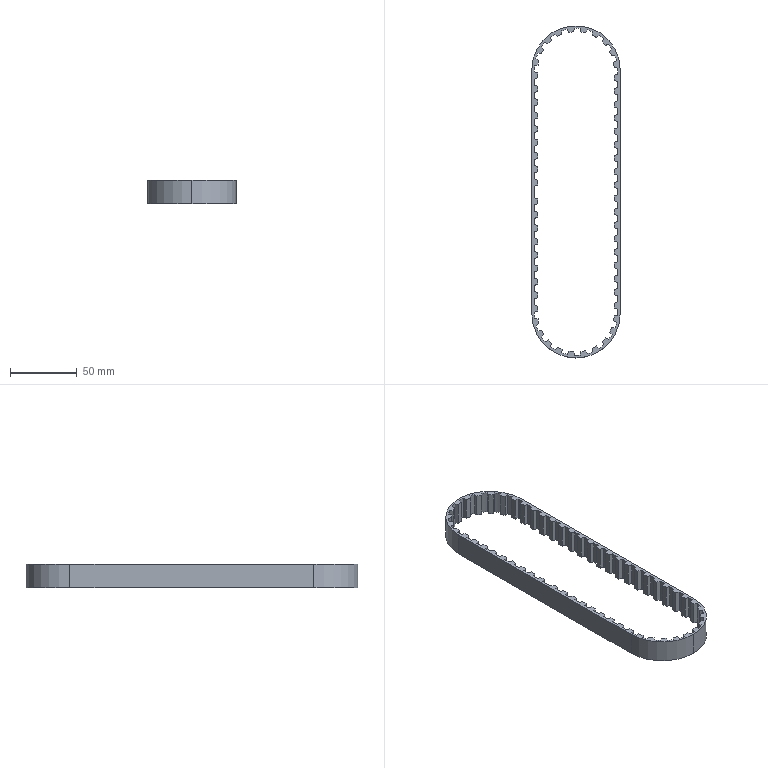Component | SolidWorks | SynchronousBelt-2 | 1 solid | 236 faces | box 66 x 248 x 17.3 mm | volume 30311 mm3 | plane 210 | cylinder 26 | commonest cylinder face diameters 62.1 x23 66 x3
build123d program:
from build123d import *

# Parameters (mm, degrees)
BOSS_EXTRUDE1_DEPTH                        = 17.3
T10_TOOTH_PROFILE_INNER_CONTOUR_DEPTH      = 129.624
T10_TOOTH_PROFILE_INNER_CONTOUR_DEPTH_BACK = 129.624


with BuildPart() as part:
    # Sketch1_2 → Boss-Extrude1 (new body)
    with BuildSketch(Plane.XY.offset(8.4)):
        with BuildLine():
            Line((-91, -33), (91, -33))
            ThreePointArc((91, -33), (124, 0), (91, 33))
            Line((91, 33), (-91, 33))
            ThreePointArc((-91, 33), (-124, 0), (-91, -33))
        make_face()
        with BuildLine():
            Line((-102.801, 22.266), (-102.873, 24.877))
            Line((-102.873, 24.877), (-99.358, 26.267))
            Line((-99.358, 26.267), (-97.625, 24.314))
            ThreePointArc((-97.625, 24.314), (-95.718, 24.754), (-93.783, 25.046))
            Line((-93.783, 25.046), (-92.89, 27.5))
            Line((-92.89, 27.5), (-89.11, 27.5))
            Line((-89.11, 27.5), (-88.273, 25.2))
            Line((-88.273, 25.2), (-82.803, 25.2))
            Line((-82.803, 25.2), (-81.966, 27.5))
            Line((-81.966, 27.5), (-78.186, 27.5))
            Line((-78.186, 27.5), (-77.349, 25.2))
            Line((-77.349, 25.2), (-71.879, 25.2))
            Line((-71.879, 25.2), (-71.042, 27.5))
            Line((-71.042, 27.5), (-67.261, 27.5))
            Line((-67.261, 27.5), (-66.424, 25.2))
            Line((-66.424, 25.2), (-60.954, 25.2))
            Line((-60.954, 25.2), (-60.117, 27.5))
            Line((-60.117, 27.5), (-56.337, 27.5))
            Line((-56.337, 27.5), (-55.5, 25.2))
            Line((-55.5, 25.2), (-50.03, 25.2))
            Line((-50.03, 25.2), (-49.193, 27.5))
            Line((-49.193, 27.5), (-45.413, 27.5))
            Line((-45.413, 27.5), (-44.576, 25.2))
            Line((-44.576, 25.2), (-39.106, 25.2))
            Line((-39.106, 25.2), (-38.269, 27.5))
            Line((-38.269, 27.5), (-34.489, 27.5))
            Line((-34.489, 27.5), (-33.652, 25.2))
            Line((-33.652, 25.2), (-28.182, 25.2))
            Line((-28.182, 25.2), (-27.345, 27.5))
            Line((-27.345, 27.5), (-23.564, 27.5))
            Line((-23.564, 27.5), (-22.727, 25.2))
            Line((-22.727, 25.2), (-17.257, 25.2))
            Line((-17.257, 25.2), (-16.42, 27.5))
            Line((-16.42, 27.5), (-12.64, 27.5))
            Line((-12.64, 27.5), (-11.803, 25.2))
            Line((-11.803, 25.2), (-6.333, 25.2))
            Line((-6.333, 25.2), (-5.496, 27.5))
            Line((-5.496, 27.5), (-1.716, 27.5))
            Line((-1.716, 27.5), (-0.8788, 25.2))
            Line((-0.8788, 25.2), (4.591, 25.2))
            Line((4.591, 25.2), (5.428, 27.5))
            Line((5.428, 27.5), (9.208, 27.5))
            Line((9.208, 27.5), (10.045, 25.2))
            Line((10.045, 25.2), (15.515, 25.2))
            Line((15.515, 25.2), (16.352, 27.5))
            Line((16.352, 27.5), (20.133, 27.5))
            Line((20.133, 27.5), (20.97, 25.2))
            Line((20.97, 25.2), (26.44, 25.2))
            Line((26.44, 25.2), (27.277, 27.5))
            Line((27.277, 27.5), (31.057, 27.5))
            Line((31.057, 27.5), (31.894, 25.2))
            Line((31.894, 25.2), (37.364, 25.2))
            Line((37.364, 25.2), (38.201, 27.5))
            Line((38.201, 27.5), (41.981, 27.5))
            Line((41.981, 27.5), (42.818, 25.2))
            Line((42.818, 25.2), (48.288, 25.2))
            Line((48.288, 25.2), (49.125, 27.5))
            Line((49.125, 27.5), (52.905, 27.5))
            Line((52.905, 27.5), (53.742, 25.2))
            Line((53.742, 25.2), (59.212, 25.2))
            Line((59.212, 25.2), (60.049, 27.5))
            Line((60.049, 27.5), (63.83, 27.5))
            Line((63.83, 27.5), (64.667, 25.2))
            Line((64.667, 25.2), (70.137, 25.2))
            Line((70.137, 25.2), (70.974, 27.5))
            Line((70.974, 27.5), (74.754, 27.5))
            Line((74.754, 27.5), (75.591, 25.2))
            Line((75.591, 25.2), (81.061, 25.2))
            Line((81.061, 25.2), (81.898, 27.5))
            Line((81.898, 27.5), (85.678, 27.5))
            Line((85.678, 27.5), (86.515, 25.2))
            Line((86.515, 25.2), (91, 25.2))
            ThreePointArc((91, 25.2), (91.218, 25.199), (91.437, 25.196))
            Line((91.437, 25.196), (92.636, 27.516))
            Line((92.636, 27.516), (96.385, 27.034))
            Line((96.385, 27.034), (96.958, 24.486))
            ThreePointArc((96.958, 24.486), (98.84, 23.949), (100.675, 23.269))
            Line((100.675, 23.269), (102.643, 24.985))
            Line((102.643, 24.985), (105.952, 23.157))
            Line((105.952, 23.157), (105.547, 20.577))
            ThreePointArc((105.547, 20.577), (107.1, 19.386), (108.556, 18.079))
            Line((108.556, 18.079), (111.018, 18.95))
            Line((111.018, 18.95), (113.422, 16.033))
            Line((113.422, 16.033), (112.097, 13.783))
            ThreePointArc((112.097, 13.783), (113.102, 12.105), (113.975, 10.353))
            Line((113.975, 10.353), (116.585, 10.258))
            Line((116.585, 10.258), (117.748, 6.661))
            Line((117.748, 6.661), (115.688, 5.056))
            ThreePointArc((115.688, 5.056), (116.005, 3.125), (116.173, 1.176))
            Line((116.173, 1.176), (118.565, 0.1273))
            Line((118.565, 0.1273), (118.323, -3.645))
            Line((118.323, -3.645), (115.817, -4.38))
            ThreePointArc((115.817, -4.38), (115.402, -6.292), (114.84, -8.167))
            Line((114.84, -8.167), (116.679, -10.021))
            Line((116.679, -10.021), (115.066, -13.44))
            Line((115.066, -13.44), (112.465, -13.201))
            ThreePointArc((112.465, -13.201), (111.376, -14.827), (110.164, -16.364))
            Line((110.164, -16.364), (111.192, -18.765))
            Line((111.192, -18.765), (108.435, -21.351))
            Line((108.435, -21.351), (106.104, -20.172))
            ThreePointArc((106.104, -20.172), (104.493, -21.283), (102.801, -22.266))
            Line((102.801, -22.266), (102.873, -24.877))
            Line((102.873, -24.877), (99.358, -26.267))
            Line((99.358, -26.267), (97.625, -24.314))
            ThreePointArc((97.625, -24.314), (95.718, -24.754), (93.783, -25.046))
            Line((93.783, -25.046), (92.89, -27.5))
            Line((92.89, -27.5), (89.11, -27.5))
            Line((89.11, -27.5), (88.273, -25.2))
            Line((88.273, -25.2), (82.803, -25.2))
            Line((82.803, -25.2), (81.966, -27.5))
            Line((81.966, -27.5), (78.186, -27.5))
            Line((78.186, -27.5), (77.349, -25.2))
            Line((77.349, -25.2), (71.879, -25.2))
            Line((71.879, -25.2), (71.042, -27.5))
            Line((71.042, -27.5), (67.261, -27.5))
            Line((67.261, -27.5), (66.424, -25.2))
            Line((66.424, -25.2), (60.954, -25.2))
            Line((60.954, -25.2), (60.117, -27.5))
            Line((60.117, -27.5), (56.337, -27.5))
            Line((56.337, -27.5), (55.5, -25.2))
            Line((55.5, -25.2), (50.03, -25.2))
            Line((50.03, -25.2), (49.193, -27.5))
            Line((49.193, -27.5), (45.413, -27.5))
            Line((45.413, -27.5), (44.576, -25.2))
            Line((44.576, -25.2), (39.106, -25.2))
            Line((39.106, -25.2), (38.269, -27.5))
            Line((38.269, -27.5), (34.489, -27.5))
            Line((34.489, -27.5), (33.652, -25.2))
            Line((33.652, -25.2), (28.182, -25.2))
            Line((28.182, -25.2), (27.345, -27.5))
            Line((27.345, -27.5), (23.564, -27.5))
            Line((23.564, -27.5), (22.727, -25.2))
            Line((22.727, -25.2), (17.257, -25.2))
            Line((17.257, -25.2), (16.42, -27.5))
            Line((16.42, -27.5), (12.64, -27.5))
            Line((12.64, -27.5), (11.803, -25.2))
            Line((11.803, -25.2), (6.333, -25.2))
            Line((6.333, -25.2), (5.496, -27.5))
            Line((5.496, -27.5), (1.716, -27.5))
            Line((1.716, -27.5), (0.8788, -25.2))
            Line((0.8788, -25.2), (-4.591, -25.2))
            Line((-4.591, -25.2), (-5.428, -27.5))
            Line((-5.428, -27.5), (-9.208, -27.5))
            Line((-9.208, -27.5), (-10.045, -25.2))
            Line((-10.045, -25.2), (-15.515, -25.2))
            Line((-15.515, -25.2), (-16.352, -27.5))
            Line((-16.352, -27.5), (-20.133, -27.5))
            Line((-20.133, -27.5), (-20.97, -25.2))
            Line((-20.97, -25.2), (-26.44, -25.2))
            Line((-26.44, -25.2), (-27.277, -27.5))
            Line((-27.277, -27.5), (-31.057, -27.5))
            Line((-31.057, -27.5), (-31.894, -25.2))
            Line((-31.894, -25.2), (-37.364, -25.2))
            Line((-37.364, -25.2), (-38.201, -27.5))
            Line((-38.201, -27.5), (-41.981, -27.5))
            Line((-41.981, -27.5), (-42.818, -25.2))
            Line((-42.818, -25.2), (-48.288, -25.2))
            Line((-48.288, -25.2), (-49.125, -27.5))
            Line((-49.125, -27.5), (-52.905, -27.5))
            Line((-52.905, -27.5), (-53.742, -25.2))
            Line((-53.742, -25.2), (-59.212, -25.2))
            Line((-59.212, -25.2), (-60.049, -27.5))
            Line((-60.049, -27.5), (-63.83, -27.5))
            Line((-63.83, -27.5), (-64.667, -25.2))
            Line((-64.667, -25.2), (-70.137, -25.2))
            Line((-70.137, -25.2), (-70.974, -27.5))
            Line((-70.974, -27.5), (-74.754, -27.5))
            Line((-74.754, -27.5), (-75.591, -25.2))
            Line((-75.591, -25.2), (-81.061, -25.2))
            Line((-81.061, -25.2), (-81.898, -27.5))
            Line((-81.898, -27.5), (-85.678, -27.5))
            Line((-85.678, -27.5), (-86.515, -25.2))
            Line((-86.515, -25.2), (-91, -25.2))
            ThreePointArc((-91, -25.2), (-91.218, -25.199), (-91.437, -25.196))
            Line((-91.437, -25.196), (-92.636, -27.516))
            Line((-92.636, -27.516), (-96.385, -27.034))
            Line((-96.385, -27.034), (-96.958, -24.486))
            ThreePointArc((-96.958, -24.486), (-98.84, -23.949), (-100.675, -23.269))
            Line((-100.675, -23.269), (-102.643, -24.985))
            Line((-102.643, -24.985), (-105.952, -23.157))
            Line((-105.952, -23.157), (-105.547, -20.577))
            ThreePointArc((-105.547, -20.577), (-107.1, -19.386), (-108.556, -18.079))
            Line((-108.556, -18.079), (-111.018, -18.95))
            Line((-111.018, -18.95), (-113.422, -16.033))
            Line((-113.422, -16.033), (-112.097, -13.783))
            ThreePointArc((-112.097, -13.783), (-113.102, -12.105), (-113.975, -10.353))
            Line((-113.975, -10.353), (-116.585, -10.258))
            Line((-116.585, -10.258), (-117.748, -6.661))
            Line((-117.748, -6.661), (-115.688, -5.056))
            ThreePointArc((-115.688, -5.056), (-116.005, -3.125), (-116.173, -1.176))
            Line((-116.173, -1.176), (-118.565, -0.1273))
            Line((-118.565, -0.1273), (-118.323, 3.645))
            Line((-118.323, 3.645), (-115.817, 4.38))
            ThreePointArc((-115.817, 4.38), (-115.402, 6.292), (-114.84, 8.167))
            Line((-114.84, 8.167), (-116.679, 10.021))
            Line((-116.679, 10.021), (-115.066, 13.44))
            Line((-115.066, 13.44), (-112.465, 13.201))
            ThreePointArc((-112.465, 13.201), (-111.376, 14.827), (-110.164, 16.364))
            Line((-110.164, 16.364), (-111.192, 18.765))
            Line((-111.192, 18.765), (-108.435, 21.351))
            Line((-108.435, 21.351), (-106.104, 20.172))
            ThreePointArc((-106.104, 20.172), (-104.493, 21.283), (-102.801, 22.266))
        make_face(mode=Mode.SUBTRACT)
    extrude(amount=-BOSS_EXTRUDE1_DEPTH)

    # Sketch1 → T10 Tooth Profile - Inner Contour (cut, two sides: drawn at the far end of the back side and taken through both)
    with BuildSketch(Plane.XY.offset(-T10_TOOTH_PROFILE_INNER_CONTOUR_DEPTH_BACK)):
        with BuildLine():
            Line((94.235, -30.881), (94.623, -28.329))
            Line((94.623, -28.329), (98.255, -27.623))
            Line((98.255, -27.623), (99.569, -29.844))
            ThreePointArc((99.569, -29.844), (101.62, -29.177), (103.62, -28.37))
            Line((103.62, -28.37), (103.199, -25.823))
            Line((103.199, -25.823), (106.436, -24.029))
            Line((106.436, -24.029), (108.372, -25.735))
            ThreePointArc((108.372, -25.735), (110.117, -24.467), (111.769, -23.082))
            Line((111.769, -23.082), (110.582, -20.79))
            Line((110.582, -20.79), (113.106, -18.084))
            Line((113.106, -18.084), (115.475, -19.107))
            ThreePointArc((115.475, -19.107), (116.742, -17.362), (117.885, -15.534))
            Line((117.885, -15.534), (116.048, -13.721))
            Line((116.048, -13.721), (117.612, -10.367))
            Line((117.612, -10.367), (120.181, -10.609))
            ThreePointArc((120.181, -10.609), (120.847, -8.558), (121.369, -6.466))
            Line((121.369, -6.466), (119.062, -5.309))
            Line((119.062, -5.309), (119.513, -1.637))
            Line((119.513, -1.637), (122.031, -1.072))
            ThreePointArc((122.031, -1.072), (122.031, 1.084), (121.881, 3.235))
            Line((121.881, 3.235), (119.329, 3.623))
            Line((119.329, 3.623), (118.623, 7.255))
            Line((118.623, 7.255), (120.844, 8.569))
            ThreePointArc((120.844, 8.569), (120.177, 10.62), (119.37, 12.62))
            Line((119.37, 12.62), (116.823, 12.199))
            Line((116.823, 12.199), (115.029, 15.436))
            Line((115.029, 15.436), (116.735, 17.372))
            ThreePointArc((116.735, 17.372), (115.467, 19.117), (114.082, 20.769))
            Line((114.082, 20.769), (111.79, 19.582))
            Line((111.79, 19.582), (109.084, 22.106))
            Line((109.084, 22.106), (110.107, 24.475))
            ThreePointArc((110.107, 24.475), (108.362, 25.742), (106.534, 26.885))
            Line((106.534, 26.885), (104.721, 25.048))
            Line((104.721, 25.048), (101.367, 26.612))
            Line((101.367, 26.612), (101.609, 29.181))
            ThreePointArc((101.609, 29.181), (99.558, 29.847), (97.466, 30.369))
            Line((97.466, 30.369), (96.309, 28.062))
            Line((96.309, 28.062), (92.637, 28.513))
            Line((92.637, 28.513), (92.072, 31.031))
            ThreePointArc((92.072, 31.031), (91.536, 31.045), (91, 31.05))
            Line((91, 31.05), (87.605, 31.05))
            Line((87.605, 31.05), (86.738, 28.5))
            Line((86.738, 28.5), (83.038, 28.5))
            Line((83.038, 28.5), (82.171, 31.05))
            Line((82.171, 31.05), (77.605, 31.05))
            Line((77.605, 31.05), (76.738, 28.5))
            Line((76.738, 28.5), (73.038, 28.5))
            Line((73.038, 28.5), (72.171, 31.05))
            Line((72.171, 31.05), (67.605, 31.05))
            Line((67.605, 31.05), (66.738, 28.5))
            Line((66.738, 28.5), (63.038, 28.5))
            Line((63.038, 28.5), (62.171, 31.05))
            Line((62.171, 31.05), (57.605, 31.05))
            Line((57.605, 31.05), (56.738, 28.5))
            Line((56.738, 28.5), (53.038, 28.5))
            Line((53.038, 28.5), (52.171, 31.05))
            Line((52.171, 31.05), (47.605, 31.05))
            Line((47.605, 31.05), (46.738, 28.5))
            Line((46.738, 28.5), (43.038, 28.5))
            Line((43.038, 28.5), (42.171, 31.05))
            Line((42.171, 31.05), (37.605, 31.05))
            Line((37.605, 31.05), (36.738, 28.5))
            Line((36.738, 28.5), (33.038, 28.5))
            Line((33.038, 28.5), (32.171, 31.05))
            Line((32.171, 31.05), (27.605, 31.05))
            Line((27.605, 31.05), (26.738, 28.5))
            Line((26.738, 28.5), (23.038, 28.5))
            Line((23.038, 28.5), (22.171, 31.05))
            Line((22.171, 31.05), (17.605, 31.05))
            Line((17.605, 31.05), (16.738, 28.5))
            Line((16.738, 28.5), (13.038, 28.5))
            Line((13.038, 28.5), (12.171, 31.05))
            Line((12.171, 31.05), (7.605, 31.05))
            Line((7.605, 31.05), (6.738, 28.5))
            Line((6.738, 28.5), (3.038, 28.5))
            Line((3.038, 28.5), (2.171, 31.05))
            Line((2.171, 31.05), (-2.395, 31.05))
            Line((-2.395, 31.05), (-3.262, 28.5))
            Line((-3.262, 28.5), (-6.962, 28.5))
            Line((-6.962, 28.5), (-7.829, 31.05))
            Line((-7.829, 31.05), (-12.395, 31.05))
            Line((-12.395, 31.05), (-13.262, 28.5))
            Line((-13.262, 28.5), (-16.962, 28.5))
            Line((-16.962, 28.5), (-17.829, 31.05))
            Line((-17.829, 31.05), (-22.395, 31.05))
            Line((-22.395, 31.05), (-23.262, 28.5))
            Line((-23.262, 28.5), (-26.962, 28.5))
            Line((-26.962, 28.5), (-27.829, 31.05))
            Line((-27.829, 31.05), (-32.395, 31.05))
            Line((-32.395, 31.05), (-33.262, 28.5))
            Line((-33.262, 28.5), (-36.962, 28.5))
            Line((-36.962, 28.5), (-37.829, 31.05))
            Line((-37.829, 31.05), (-42.395, 31.05))
            Line((-42.395, 31.05), (-43.262, 28.5))
            Line((-43.262, 28.5), (-46.962, 28.5))
            Line((-46.962, 28.5), (-47.829, 31.05))
            Line((-47.829, 31.05), (-52.395, 31.05))
            Line((-52.395, 31.05), (-53.262, 28.5))
            Line((-53.262, 28.5), (-56.962, 28.5))
            Line((-56.962, 28.5), (-57.829, 31.05))
            Line((-57.829, 31.05), (-62.395, 31.05))
            Line((-62.395, 31.05), (-63.262, 28.5))
            Line((-63.262, 28.5), (-66.962, 28.5))
            Line((-66.962, 28.5), (-67.829, 31.05))
            Line((-67.829, 31.05), (-72.395, 31.05))
            Line((-72.395, 31.05), (-73.262, 28.5))
            Line((-73.262, 28.5), (-76.962, 28.5))
            Line((-76.962, 28.5), (-77.829, 31.05))
            Line((-77.829, 31.05), (-82.395, 31.05))
            Line((-82.395, 31.05), (-83.262, 28.5))
            Line((-83.262, 28.5), (-86.962, 28.5))
            Line((-86.962, 28.5), (-87.829, 31.05))
            Line((-87.829, 31.05), (-91, 31.05))
            ThreePointArc((-91, 31.05), (-91.644, 31.043), (-92.287, 31.023))
            Line((-92.287, 31.023), (-92.834, 28.501))
            Line((-92.834, 28.501), (-96.503, 28.025))
            Line((-96.503, 28.025), (-97.676, 30.324))
            ThreePointArc((-97.676, 30.324), (-99.765, 29.787), (-101.811, 29.107))
            Line((-101.811, 29.107), (-101.552, 26.539))
            Line((-101.552, 26.539), (-104.894, 24.952))
            Line((-104.894, 24.952), (-106.72, 26.777))
            ThreePointArc((-106.72, 26.777), (-108.54, 25.621), (-110.276, 24.342))
            Line((-110.276, 24.342), (-109.236, 21.98))
            Line((-109.236, 21.98), (-111.925, 19.438))
            Line((-111.925, 19.438), (-114.225, 20.608))
            ThreePointArc((-114.225, 20.608), (-115.599, 18.947), (-116.855, 17.194))
            Line((-116.855, 17.194), (-115.136, 15.269))
            Line((-115.136, 15.269), (-116.907, 12.02))
            Line((-116.907, 12.02), (-119.457, 12.423))
            ThreePointArc((-119.457, 12.423), (-120.25, 10.418), (-120.903, 8.363))
            Line((-120.903, 8.363), (-118.673, 7.063))
            Line((-118.673, 7.063), (-119.354, 3.426))
            Line((-119.354, 3.426), (-121.903, 3.021))
            ThreePointArc((-121.903, 3.021), (-122.038, 0.8691), (-122.023, -1.287))
            Line((-122.023, -1.287), (-119.501, -1.834))
            Line((-119.501, -1.834), (-119.025, -5.503))
            Line((-119.025, -5.503), (-121.324, -6.676))
            ThreePointArc((-121.324, -6.676), (-120.787, -8.765), (-120.107, -10.811))
            Line((-120.107, -10.811), (-117.539, -10.552))
            Line((-117.539, -10.552), (-115.952, -13.894))
            Line((-115.952, -13.894), (-117.777, -15.72))
            ThreePointArc((-117.777, -15.72), (-116.621, -17.54), (-115.342, -19.276))
            Line((-115.342, -19.276), (-112.98, -18.236))
            Line((-112.98, -18.236), (-110.438, -20.925))
            Line((-110.438, -20.925), (-111.608, -23.225))
            ThreePointArc((-111.608, -23.225), (-109.947, -24.599), (-108.194, -25.855))
            Line((-108.194, -25.855), (-106.269, -24.136))
            Line((-106.269, -24.136), (-103.02, -25.907))
            Line((-103.02, -25.907), (-103.423, -28.457))
            ThreePointArc((-103.423, -28.457), (-101.418, -29.25), (-99.363, -29.903))
            Line((-99.363, -29.903), (-98.063, -27.673))
            Line((-98.063, -27.673), (-94.426, -28.354))
            Line((-94.426, -28.354), (-94.021, -30.903))
            ThreePointArc((-94.021, -30.903), (-92.512, -31.013), (-91, -31.05))
            Line((-91, -31.05), (-89.608, -31.05))
            Line((-89.608, -31.05), (-88.741, -28.5))
            Line((-88.741, -28.5), (-85.041, -28.5))
            Line((-85.041, -28.5), (-84.174, -31.05))
            Line((-84.174, -31.05), (-79.608, -31.05))
            Line((-79.608, -31.05), (-78.741, -28.5))
            Line((-78.741, -28.5), (-75.041, -28.5))
            Line((-75.041, -28.5), (-74.174, -31.05))
            Line((-74.174, -31.05), (-69.608, -31.05))
            Line((-69.608, -31.05), (-68.741, -28.5))
            Line((-68.741, -28.5), (-65.041, -28.5))
            Line((-65.041, -28.5), (-64.174, -31.05))
            Line((-64.174, -31.05), (-59.608, -31.05))
            Line((-59.608, -31.05), (-58.741, -28.5))
            Line((-58.741, -28.5), (-55.041, -28.5))
            Line((-55.041, -28.5), (-54.174, -31.05))
            Line((-54.174, -31.05), (-49.608, -31.05))
            Line((-49.608, -31.05), (-48.741, -28.5))
            Line((-48.741, -28.5), (-45.041, -28.5))
            Line((-45.041, -28.5), (-44.174, -31.05))
            Line((-44.174, -31.05), (-39.608, -31.05))
            Line((-39.608, -31.05), (-38.741, -28.5))
            Line((-38.741, -28.5), (-35.041, -28.5))
            Line((-35.041, -28.5), (-34.174, -31.05))
            Line((-34.174, -31.05), (-29.608, -31.05))
            Line((-29.608, -31.05), (-28.741, -28.5))
            Line((-28.741, -28.5), (-25.041, -28.5))
            Line((-25.041, -28.5), (-24.174, -31.05))
            Line((-24.174, -31.05), (-19.608, -31.05))
            Line((-19.608, -31.05), (-18.741, -28.5))
            Line((-18.741, -28.5), (-15.041, -28.5))
            Line((-15.041, -28.5), (-14.174, -31.05))
            Line((-14.174, -31.05), (-9.608, -31.05))
            Line((-9.608, -31.05), (-8.741, -28.5))
            Line((-8.741, -28.5), (-5.041, -28.5))
            Line((-5.041, -28.5), (-4.174, -31.05))
            Line((-4.174, -31.05), (4.394, -31.05))
            Line((4.394, -31.05), (5.261, -28.5))
            Line((5.261, -28.5), (8.961, -28.5))
            Line((8.961, -28.5), (9.828, -31.05))
            Line((9.828, -31.05), (14.394, -31.05))
            Line((14.394, -31.05), (15.261, -28.5))
            Line((15.261, -28.5), (18.961, -28.5))
            Line((18.961, -28.5), (19.828, -31.05))
            Line((19.828, -31.05), (24.394, -31.05))
            Line((24.394, -31.05), (25.261, -28.5))
            Line((25.261, -28.5), (28.961, -28.5))
            Line((28.961, -28.5), (29.828, -31.05))
            Line((29.828, -31.05), (34.394, -31.05))
            Line((34.394, -31.05), (35.261, -28.5))
            Line((35.261, -28.5), (38.961, -28.5))
            Line((38.961, -28.5), (39.828, -31.05))
            Line((39.828, -31.05), (44.394, -31.05))
            Line((44.394, -31.05), (45.261, -28.5))
            Line((45.261, -28.5), (48.961, -28.5))
            Line((48.961, -28.5), (49.828, -31.05))
            Line((49.828, -31.05), (54.394, -31.05))
            Line((54.394, -31.05), (55.261, -28.5))
            Line((55.261, -28.5), (58.961, -28.5))
            Line((58.961, -28.5), (59.828, -31.05))
            Line((59.828, -31.05), (64.394, -31.05))
            Line((64.394, -31.05), (65.261, -28.5))
            Line((65.261, -28.5), (68.961, -28.5))
            Line((68.961, -28.5), (69.828, -31.05))
            Line((69.828, -31.05), (74.394, -31.05))
            Line((74.394, -31.05), (75.261, -28.5))
            Line((75.261, -28.5), (78.961, -28.5))
            Line((78.961, -28.5), (79.828, -31.05))
            Line((79.828, -31.05), (84.394, -31.05))
            Line((84.394, -31.05), (85.261, -28.5))
            Line((85.261, -28.5), (88.961, -28.5))
            Line((88.961, -28.5), (89.828, -31.05))
            Line((89.828, -31.05), (91, -31.05))
            ThreePointArc((91, -31.05), (92.62, -31.008), (94.235, -30.881))
        make_face()
    extrude(amount=T10_TOOTH_PROFILE_INNER_CONTOUR_DEPTH + T10_TOOTH_PROFILE_INNER_CONTOUR_DEPTH_BACK, mode=Mode.SUBTRACT)


solid = part.part

# Placed as in the assembly
solid = solid.moved(Location((85.931, 269, 140), (0, 0, -90)))